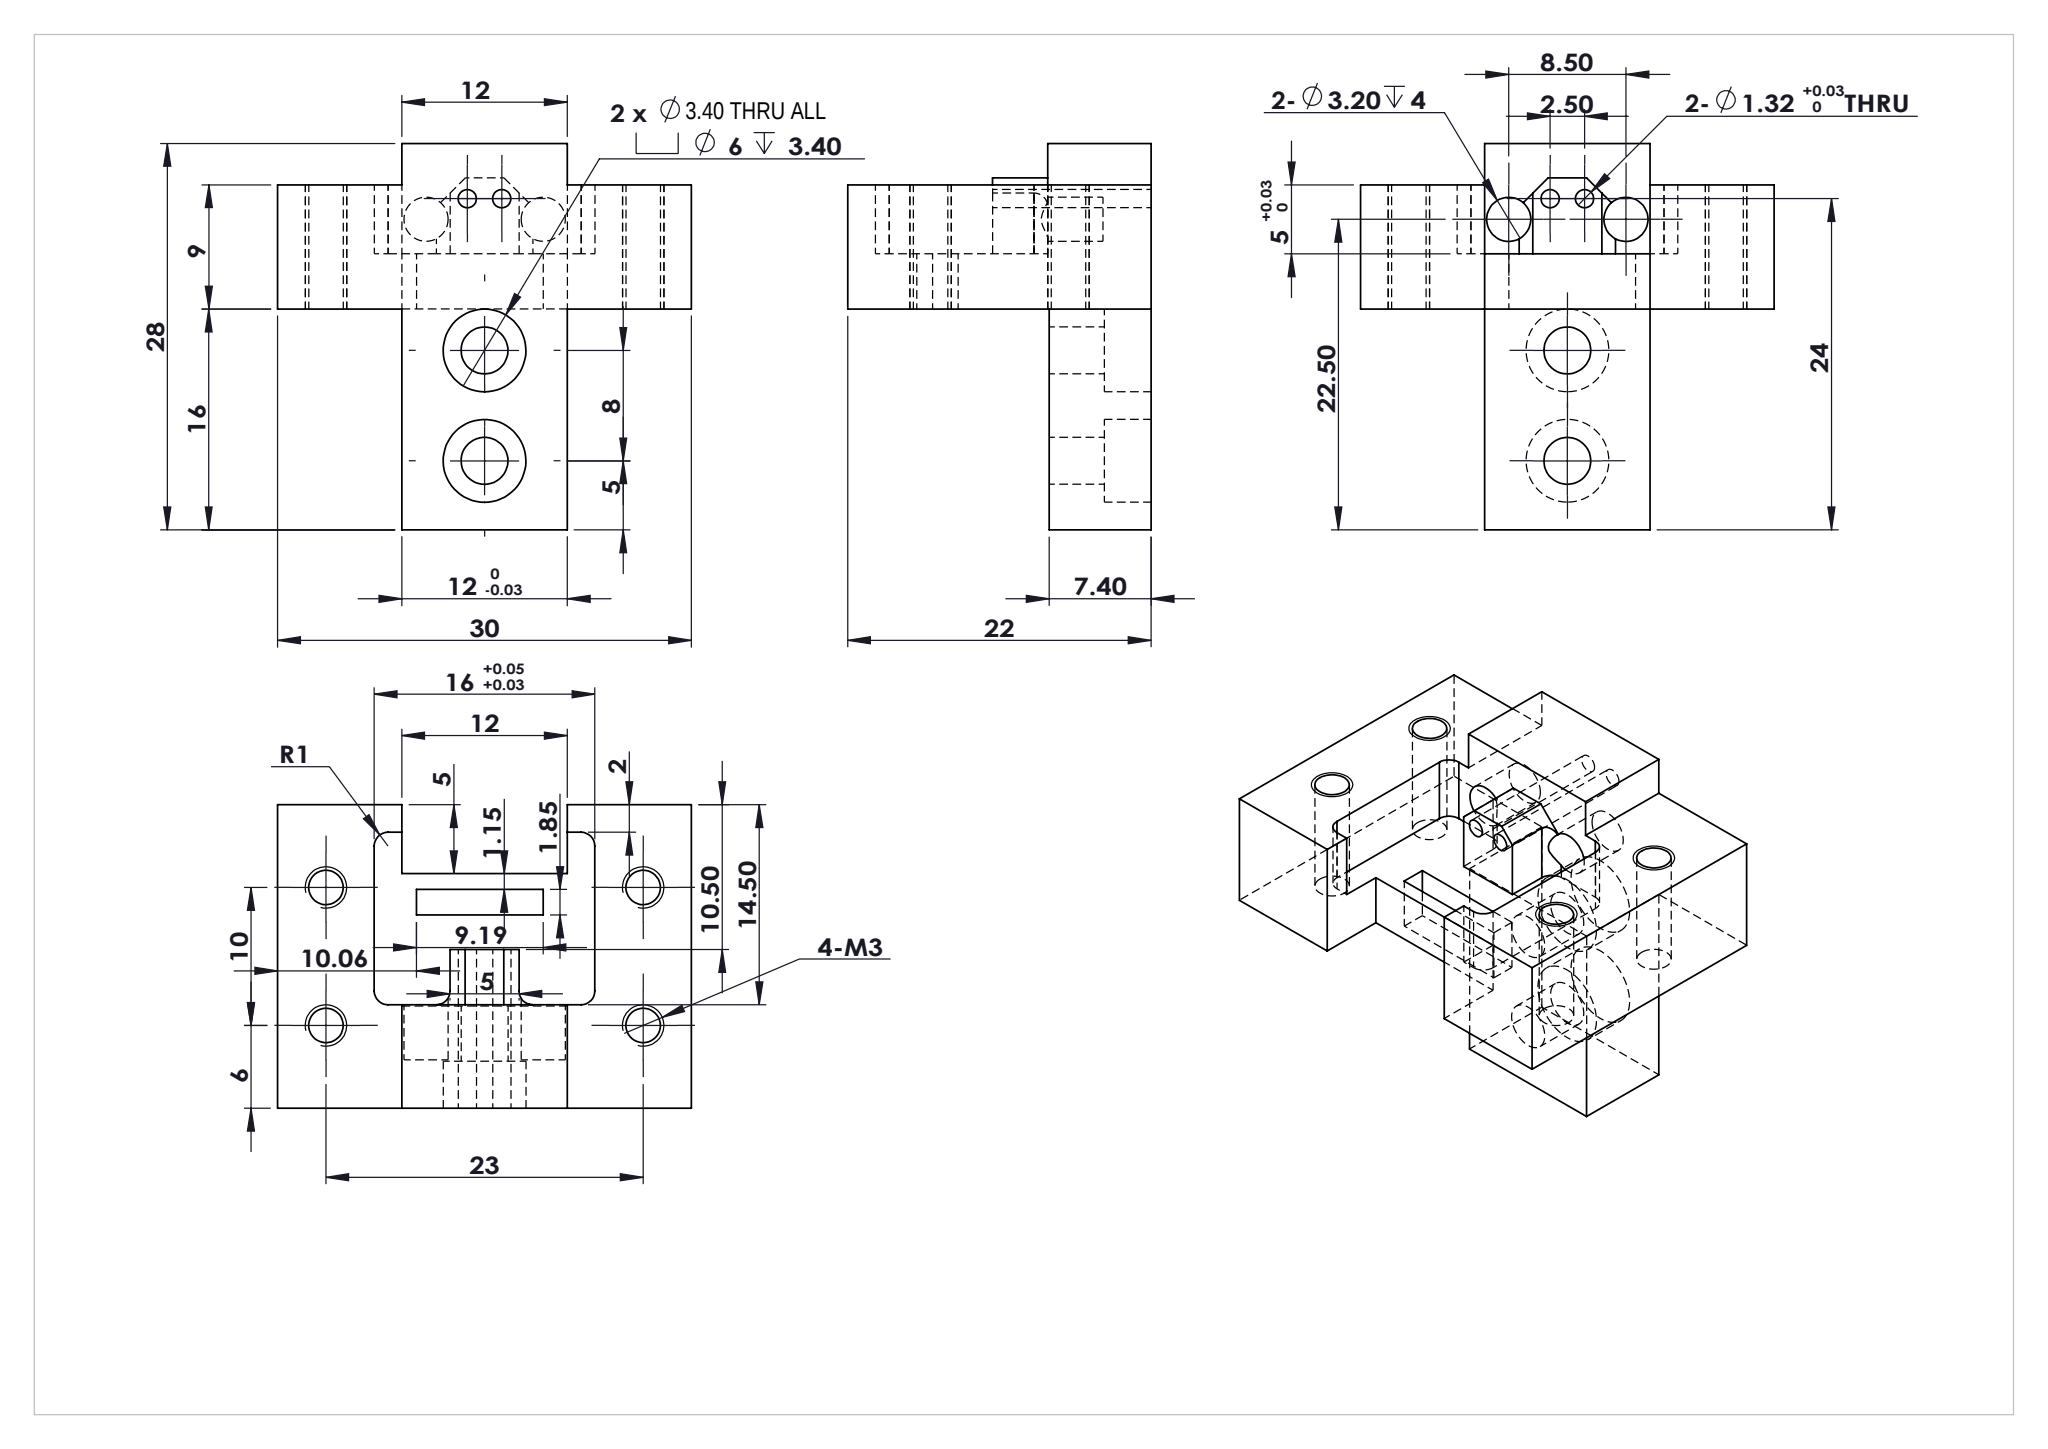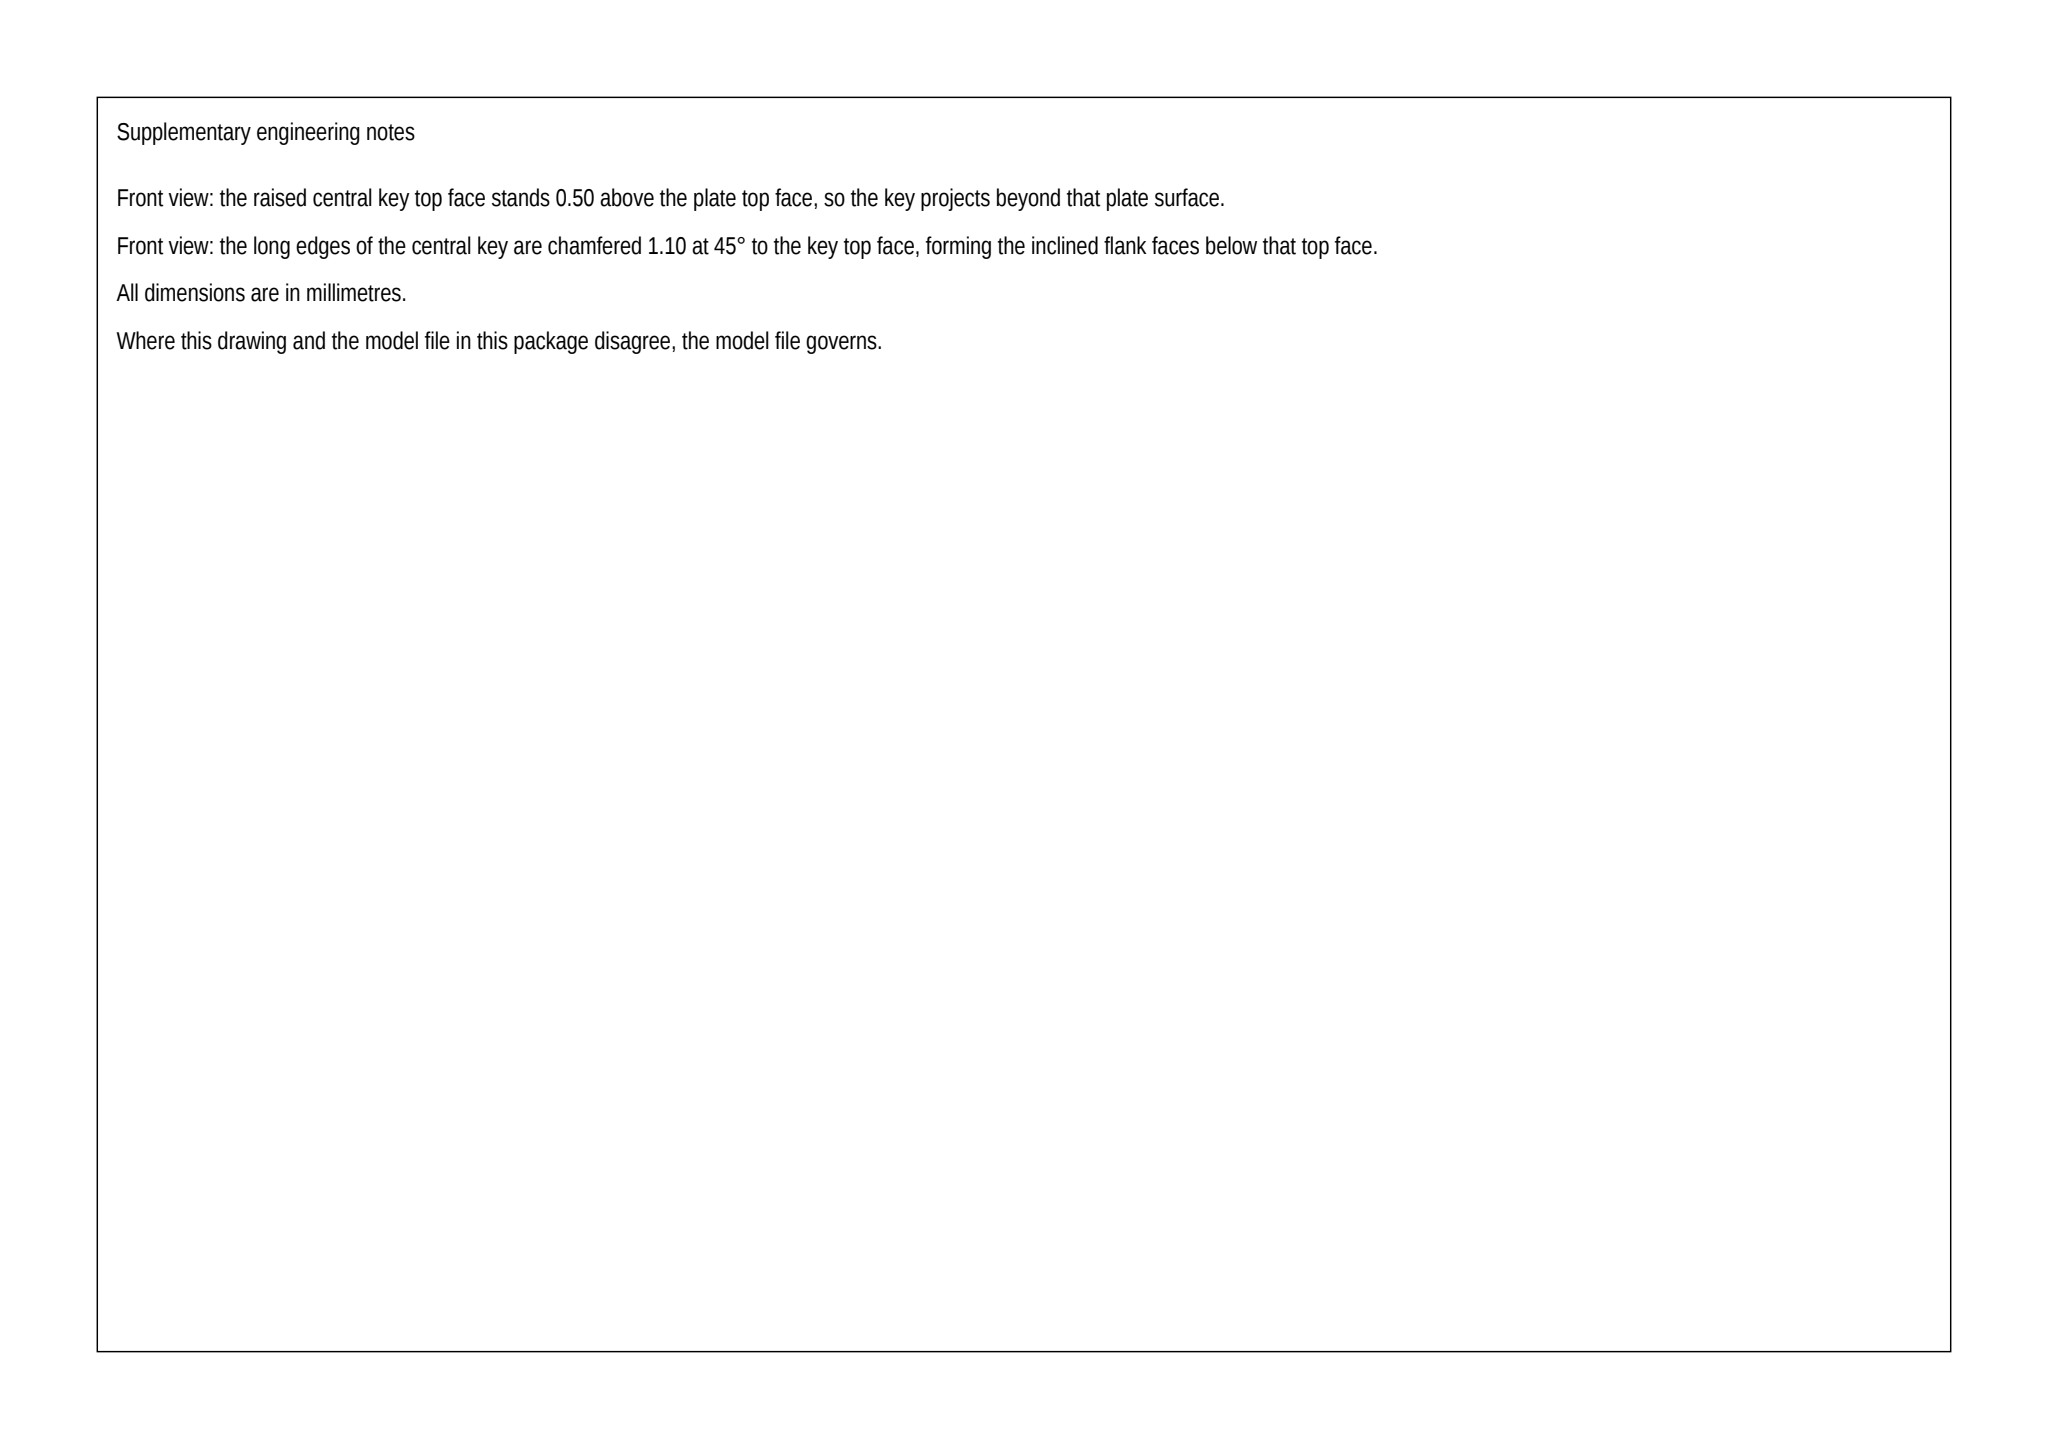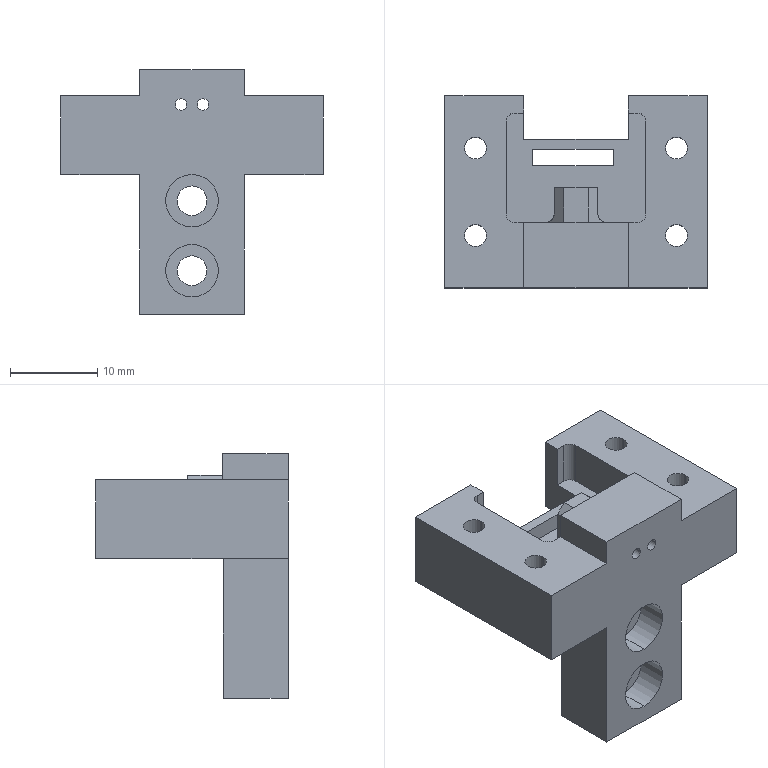Part | SolidWorks | mm | 1 solid | 68 faces | box 30 x 22 x 28 mm | volume 5776 mm3 | plane 38 | cylinder 30 | commonest cylinder face diameters 2.5 x8 2 x6 3.2 x4 6 x4 3.4 x4 1.32 x4
build123d program:
from build123d import *

# Parameters (mm, degrees)
SKETCH1_2_W                                          = 30
SKETCH1_2_H                                          = 20
BOSS_EXTRUDE1_2_DEPTH                                = 12
SKETCH2_2_W                                          = 16
SKETCH2_2_H                                          = 10.5
CUT_EXTRUDE1_2_DEPTH                                 = 8
SKETCH3_2_W                                          = 16
SKETCH3_2_H                                          = 5
CUT_EXTRUDE2_2_DEPTH                                 = 22.656
SKETCH4_2_W                                          = 2
SKETCH4_2_H                                          = 2
BOSS_EXTRUDE2_DEPTH                                  = 12
SKETCH5_2_W                                          = 12
SKETCH5_2_H                                          = 5.4
BOSS_EXTRUDE3_DEPTH                                  = 16
SKETCH1_R                                            = 0.66
CUT_EXTRUDE1_DEPTH                                   = 25.316
SKETCH3_W                                            = 2
SKETCH3_H                                            = 3
BOSS_EXTRUDE1_DEPTH                                  = 4
SKETCH8_W                                            = 9
SKETCH8_H                                            = 20
CUT_EXTRUDE3_DEPTH                                   = 3
M3_TAPPED_HOLE1_D                                    = 2.5
MOVE_FACE1_BY                                        = 2
CBORE_FOR_M3_HEXAGON_SOCKET_HEAD_CAP_SCR_D           = 3.4
CBORE_FOR_M3_HEXAGON_SOCKET_HEAD_CAP_SCR_CBORE_D     = 6
CBORE_FOR_M3_HEXAGON_SOCKET_HEAD_CAP_SCR_CBORE_DEPTH = 3.4
CUT_EXTRUDE3_2_START                                 = -8
SKETCH6_2_W                                          = 5.5
SKETCH6_2_H                                          = 4
CUT_EXTRUDE3_2_DEPTH                                 = 8
SKETCH7_2_W                                          = 5
SKETCH7_2_H                                          = 4
CUT_EXTRUDE4_DEPTH                                   = 2.5
CHAMFER1_SIZE                                        = 1.1
FILLET1_R                                            = 1
SKETCH2_R                                            = 1.6
CUT_EXTRUDE2_DEPTH                                   = 8
SKETCH8_2_W                                          = 9.187
SKETCH8_2_H                                          = 1.852
CUT_EXTRUDE5_DEPTH                                   = 10


with BuildPart() as part:
    # Sketch1_2 → Boss-Extrude1_2 (new body)
    with BuildSketch(Plane.XY):
        Rectangle(SKETCH1_2_W, SKETCH1_2_H)
    extrude(amount=BOSS_EXTRUDE1_2_DEPTH)

    # Sketch2_2 → Cut-Extrude1_2 (cut)
    with BuildSketch(Plane.XY.offset(12)):
        with Locations((0, 4.75)):
            Rectangle(SKETCH2_2_W, SKETCH2_2_H)
    extrude(amount=-CUT_EXTRUDE1_2_DEPTH, mode=Mode.SUBTRACT)

    # Sketch3_2 → Cut-Extrude2_2 (cut, through all)
    with BuildSketch(Plane.XY.offset(12)):
        with Locations((0, 7.5)):
            Rectangle(SKETCH3_2_W, SKETCH3_2_H)
    extrude(amount=-CUT_EXTRUDE2_2_DEPTH, mode=Mode.SUBTRACT)

    # Sketch4_2 → Boss-Extrude2 (add)
    with BuildSketch(Plane.XY.offset(12)):
        with Locations((-7, 9)):
            Rectangle(SKETCH4_2_W, SKETCH4_2_H)
        with Locations((7, 9)):
            Rectangle(SKETCH4_2_W, SKETCH4_2_H)
    extrude(amount=-BOSS_EXTRUDE2_DEPTH)

    # Sketch5_2 → Boss-Extrude3 (add)
    with BuildSketch(Plane(origin=(0, 0, 0), x_dir=(-1, 0, 0), z_dir=(0, 0, -1))):
        with Locations((0, -7.3)):
            Rectangle(SKETCH5_2_W, SKETCH5_2_H)
    extrude(amount=BOSS_EXTRUDE3_DEPTH)

    # Sketch1 → Cut-Extrude1 (cut, through all)
    with BuildSketch(Plane(origin=(0, -0.5, 0), x_dir=(1, 0, 0), z_dir=(0, 1, 0))):
        with Locations(Location((1.25, -8, 0), (0, 0, 180))):
            Circle(SKETCH1_R)
        with Locations(Location((-1.25, -8, 0), (0, 0, 180))):
            Circle(SKETCH1_R)
    extrude(amount=-CUT_EXTRUDE1_DEPTH, mode=Mode.SUBTRACT)

    # Sketch3 → Boss-Extrude1 (add)
    with BuildSketch(Plane.XY.offset(4)):
        with Locations((-7, 6.5)):
            Rectangle(SKETCH3_W, SKETCH3_H)
        with Locations((7, 6.5)):
            Rectangle(SKETCH3_W, SKETCH3_H)
    extrude(amount=-BOSS_EXTRUDE1_DEPTH)

    # Sketch8 → Cut-Extrude3 (cut)
    with BuildSketch(Plane.XY.offset(12)):
        with Locations((-10.5, 0)):
            Rectangle(SKETCH8_W, SKETCH8_H)
        with Locations((10.5, 0)):
            Rectangle(SKETCH8_W, SKETCH8_H)
    extrude(amount=-CUT_EXTRUDE3_DEPTH, mode=Mode.SUBTRACT)

    # M3 Tapped Hole1 (through all)
    with Locations(Plane(origin=(-11.063, -5.094, 9), x_dir=(1, 0, 0), z_dir=(0, 0, 1))):
        with Locations((22.563, -0.906), (-0.4366, -0.906), (22.563, 9.094), (-0.4366, 9.094)):
            Hole(M3_TAPPED_HOLE1_D / 2)

    # Move Face1: a face moved outward by 2.0
    extrude(part.faces().sort_by_distance((0, -10, 0.07088))[0], amount=MOVE_FACE1_BY, dir=(0, -1, 0))

    # CBORE for M3 Hexagon socket head cap scr (through all)
    with Locations(Plane(origin=(0, -12, 0), x_dir=(-1, 0, 0), z_dir=(0, -1, 0))):
        with Locations((0, 11), (0, 3)):
            CounterBoreHole(CBORE_FOR_M3_HEXAGON_SOCKET_HEAD_CAP_SCR_D / 2, CBORE_FOR_M3_HEXAGON_SOCKET_HEAD_CAP_SCR_CBORE_D / 2, CBORE_FOR_M3_HEXAGON_SOCKET_HEAD_CAP_SCR_CBORE_DEPTH)

    # Sketch6_2 → Cut-Extrude3_2 (cut)
    with BuildSketch(Plane.XY.offset(12).offset(CUT_EXTRUDE3_2_START)):
        with Locations((-5.25, -2.5)):
            Rectangle(SKETCH6_2_W, SKETCH6_2_H)
        with Locations((5.25, -2.5)):
            Rectangle(SKETCH6_2_W, SKETCH6_2_H)
    extrude(amount=CUT_EXTRUDE3_2_DEPTH, mode=Mode.SUBTRACT)

    # Sketch7_2 → Cut-Extrude4 (cut)
    with BuildSketch(Plane.XY.offset(12)):
        with Locations((0, -2.5)):
            Rectangle(SKETCH7_2_W, SKETCH7_2_H)
    extrude(amount=-CUT_EXTRUDE4_DEPTH, mode=Mode.SUBTRACT)

    # Chamfer1
    chamfer1_edges = [part.edges().sort_by_distance(p)[0] for p in [
        (-2.5, -2.5, 9.5),
        (2.5, -2.5, 9.5),
    ]]
    chamfer(chamfer1_edges, length=CHAMFER1_SIZE)

    # Fillet1
    fillet1_edges = [part.edges().sort_by_distance(p)[0] for p in [
        (8, 8, 6.5),
        (-8, -4.5, 6.5),
        (-2.5, -4.5, 6.2),
        (8, -4.5, 6.5),
        (2.5, -4.5, 6.2),
        (-8, 8, 6.5),
    ]]
    fillet(fillet1_edges, radius=FILLET1_R)

    # Sketch2 → Cut-Extrude2 (cut)
    with BuildSketch(Plane(origin=(0, -0.5, 0), x_dir=(1, 0, 0), z_dir=(0, 1, 0))):
        with Locations(Location((4.25, -6.5, 0), (0, 0, 180))):
            Circle(SKETCH2_R)
        with Locations(Location((-4.25, -6.5, 0), (0, 0, 62.047))):
            Circle(SKETCH2_R)
    extrude(amount=-CUT_EXTRUDE2_DEPTH, mode=Mode.SUBTRACT)

    # Sketch8_2 → Cut-Extrude5 (cut)
    with BuildSketch(Plane.XY.offset(4)):
        with Locations((-0.3442, 2.929)):
            Rectangle(SKETCH8_2_W, SKETCH8_2_H)
    extrude(amount=-CUT_EXTRUDE5_DEPTH, mode=Mode.SUBTRACT)


solid = part.part